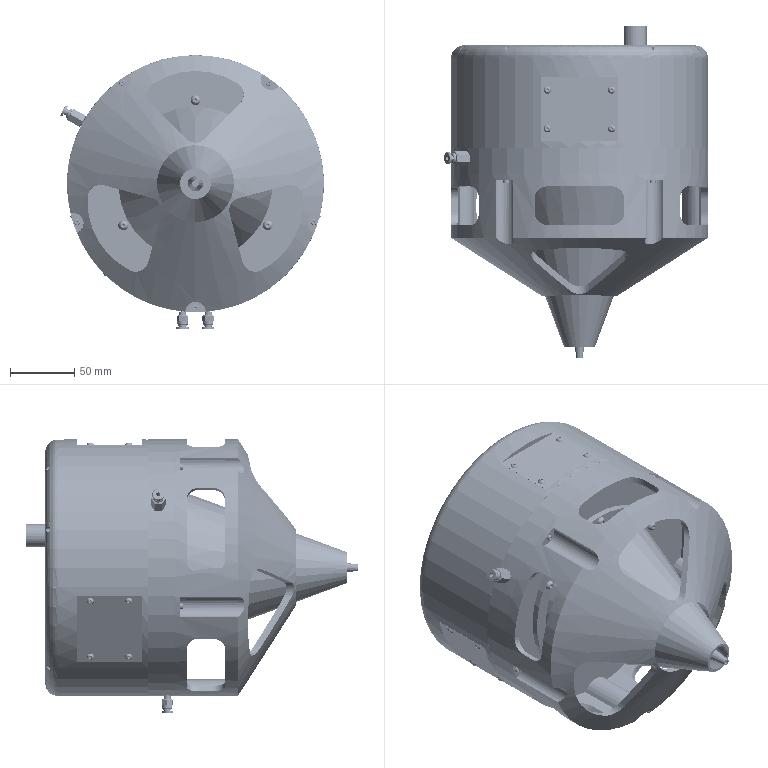Assembly | SolidWorks | mm | 111 component files | 112 solids | 5909 faces | box 205.4 x 258.5 x 213 mm | volume 1663403 mm3 | plane 2916 | cylinder 2290 | cone 400 | torus 202 | sphere 60 | spline 41 | commonest cylinder face diameters 5 x522 3 x431 7 x304 2 x192 4 x140 2.4 x66 20 x51 6 x38
Bill of materials:
AirSupplyPneumaticQuickConnectorM5 | 1 |  | Axisymmetric multi-diameter body around a hexagonal prism section. On one side of the hex is a short neck with ring/groove steps, then a thin round disk-like flange that has a central bore. On the other side is a smaller cylindrical spigot with a chamfered end and a small central hole.
CoolingPlateCover | 1 |  | Thin plain solid circular disc.
CornerCubePrism | 1 |  | Solid cylinder with one flat end and the other end cut by two inclined planes forming a ridged, roof-like end; one radial hole that appears threaded in the cylindrical wall.
CornerCubePrismCoolingPlate | 1 |  | Flanged hub: triangular plate with rounded corners and three corner through-holes, with a cylindrical boss on one side; the boss has small radial holes in its wall.
FocusingLens | 3 |  | Plain solid circular disc, thicker than a thin shim.
FocusingLensHolder | 3 |  | Square flat plate with slightly rounded corners, a large central through-hole and four smaller corner through-holes.
GB_SOCKET_TYPE7 M3X6-N | 24 |  | Headed pin: a domed (round-top) head on a plain cylindrical shank with a flat end.
GB_SOCKET_TYPE7 M4X10-N | 6 |  | Button/dome-head fastener shape with a hexagonal socket recess in the head and a plain cylindrical shank.
GB_FASTENER_SCREWS_HSHCS M2.5X6-N | 3 |  | Short cylindrical-head fastener shape: a tall round head with rounded top edge on a plain cylindrical shank with a chamfered end.
GB_FASTENER_SCREWS_HSHCS M2.5X10-N | 5 |  | Socket-head cap screw-like shape: a cylindrical head with a hexagonal socket and a cone-shaped bottom, on a long plain cylindrical shank.
GB_FASTENER_SCREWS_HSHCS M2X8-N | 2 |  | Cylindrical-head fastener shape: a round head with radiused top edge on a long plain cylindrical shank with a chamfered tip.
LaserWorkingHeadCoreComponent | 1 |  | Large circular plate with a stepped edge (reduced-diameter step on one face), three rectangular through-cutouts spaced around the center, and many small holes in the face plus at least one radial hole in the rim.
LaserWorkingHeadCover(Upper)2 | 3 |  | Flat rectangular plate with four through-holes near the corners.
LaserWorkingHeadHood(Lower) | 1 |  | Open, skeletal cup-shaped frame: cylindrical ring wall with several rounded slots, joined to a conical section that tapers to a central circular opening, with three spokes separating three large rounded windows.
Nozzle1 | 1 |  | Flanged tube: three-lobed flange with three through-holes at one end of a long cylindrical tube, with an angled wedge-like fin projecting from one side of the tube; the far end face shows a central bore surrounded by small holes.
Nozzle2 | 1 |  | Flanged tapered nozzle-like body: circular flange with three through-holes, then a cylindrical section and a conical taper ending in a small tip with a through bore; the flange side shows an internal conical cavity.
NozzleGasket1 | 1 |  | Thin three-lobed flat ring with a large central hole and a through-hole in each of the three lobes.
NozzleGasket2 | 1 |  | Flat circular ring (annular plate) with a large central hole and three equally spaced small through-holes.
Reflector | 3 |  | Solid short cylinder with one end cut off at an angle, so it ends in a wedge. A radial hole in the side wall appears threaded and has a counterbore or spot face around it.
Slider2 | 3 |  | Rectangular prismatic block with internal cylindrical passages. One passage has a stepped diameter and conical (drill-point-like) ends. The block also has a shallow groove across one face and small V-shaped notches with rounded bottoms on its edges.
Slider | 3 |  | Flat rectangular plate with rounded corners and two round through-holes. Shallow notches or grooves cross the long edges near each end. A V-shaped tab with a semicircular cutout sticks out from one long edge, and a small slot is cut into one side.
Slider3 | 3 |  | Rectangular block with a long groove on top that has angled sides, plus a narrow slit. A V-notch with a round bottom is cut into the end face. Underneath, a cylindrical or rounded boss is split by a central slot.
SliderNut1 | 3 |  | Knurled cylindrical head joined to a smaller smooth cylindrical shank. A central bore runs axially through both, and a small cross-hole passes through the shank wall.
SliderNut2 | 3 |  | Knurled cylindrical head with a smooth, smaller cylindrical shank. The visible flat end faces look solid, with no bore.
SliderScrew1 | 3 |  | Stepped cylindrical pin. A short reduced-diameter pilot is at one end, followed by a main body interrupted by a narrow circumferential groove. The other end is flat.
SliderScrew2 | 3 |  | Stepped cylindrical pin with a narrow necked groove between two equal-diameter sections. One end has a smaller-diameter cylindrical spigot.
T-Joint | 1 |  | Tubular multi-port body with three or more cylindrical ports and stepped collars at the port ends. Small ring-shaped bosses with through-holes sit beside the branch.
UpperHousing | 1 |  | Thin-walled cylindrical shell or drum with one closed end face. The end face has a large central hole, a bolt-hole pattern and small holes around a raised rim. Rectangular windows and recessed pads with small holes are cut into the side wall.
WaterPipe1 | 1 |  | Slender solid round rod bent into a curve of roughly a half-circle to three-quarters of a circle, with a short straight end section. The ends are rounded.
WaterPipe2 | 1 |  | Hollow round tube bent into a 3D path with straight runs joined by a sharp-ish bend and a roughly 90-degree radiused bend. Both ends are open and cut square.
WaterPipe3 | 1 |  | Thin-walled round tube bent into a multi-bend, roughly V/hook-shaped path, shown as two tube segments separated by a small gap along one straight run.
WaterPipe4 | 1 |  | Round tube or rod bent in three dimensions with several bends, including a sharp near-90-degree turn to one end leg.
WaterPipe5 | 1 |  | Short straight hollow cylinder (sleeve or tube section) with plain square-cut ends.
WaterPipe6 | 1 |  | Hollow round tube bent into an offset/Z-like shape: straight end leg, a long angled run, and a second bend into a short end leg.
WaterPipe7 | 1 |  | Relatively thick-walled hollow tube with several bends, including an S-curve and roughly right-angle turns.
WaterQuickConnector | 12 |  | Axially stepped turned-style body: thin circular flange disc with a large bore at one end, a grooved cylindrical collar, a hexagonal wrench-flat section, then stepped smaller cylindrical spigots ending in a small-bore tip.
WireConnectorBlock1 | 1 |  | Flat obround (stadium-shaped) plate with one large central through-hole and two smaller through-holes, one near each rounded end.
WireFeedingConnector | 1 |  | Stepped cylinder: a large-diameter main cylinder with a smaller, coaxial hollow boss sticking out from one end face, and a small central through-bore.
WireFeedingHose | 1 |  | Long, slender hollow tube that is mostly straight, with a gentle bend near one end.
WireFeedingNozzle | 1 |  | Hollow, round, spigot-like body: a long tapered section narrowing to a rounded tip, a short necked transition, a raised cylindrical collar, and a straight cylindrical end section.
WireFeedingTube | 1 |  | Hollow stepped cylindrical shaft or spacer: a long central section of larger diameter with shorter reduced-diameter sections at both ends, and a central through-bore.
WorkingHeadLowerCover | 1 |  | Thin-walled hollow cone (funnel- or hopper-like) with a flat annular flange at the large end and an open small end.
Y-Joint | 1 |  | Y-shaped tubular body. A single cylindrical branch at one end splits into two parallel cylindrical branches side by side at the other end. Every branch ends in a hollow round port with a flanged collar. A short cylindrical boss with a through-hole sits at the junction, with its hole running at right angles to the branch axes.
Mates:
1. concentric | LaserWorkingHeadCoreComponent-1 face at (-15.981, 4.506, 234.566) dir (0, 1, 0) r 2 | Slider-3 face at (-15.981, 15.849, 234.566) dir (0, 1, 0) r 1.65
2. concentric | LaserWorkingHeadCoreComponent-1 face at (4.019, 4.506, 234.566) dir (0, 1, 0) r 2 | Slider-3 face at (4.019, 15.849, 234.566) dir (0, 1, 0) r 1.65
3. coincident | LaserWorkingHeadCoreComponent-1 face at (-5.981, 10.506, 160) dir (0, 1, 0) | Slider-3 face at (-5.981, 10.506, 234.566) dir (0, -1, 0)
4. coincident | LaserWorkingHeadCoreComponent-1 face at (-5.981, 10.506, 160) dir (0, 1, 0) | Slider-4 face at (58.596, 10.506, 122.717) dir (0, -1, 0)
5. coincident | LaserWorkingHeadCoreComponent-1 face at (-5.981, 10.506, 160) dir (0, 1, 0) | Slider-5 face at (-70.557, 10.506, 122.717) dir (0, -1, 0)
6. concentric | Slider2-2 face at (68.988, 19.006, 116.717) dir (-0.866, 0, 0.5) r 1.5 | SliderScrew1-2 face at (46.471, 19.006, 129.717) dir (0.866, 0, -0.5) r 1.5
7. concentric | Slider2-3 face at (-5.981, 19.006, 246.566) dir (0, 0, -1) r 1.5 | SliderScrew1-3 face at (-5.981, 19.006, 220.566) dir (0, 0, 1) r 1.5
8. concentric | Slider2-3 face at (-20.981, 33.561, 233.566) dir (1, 0, 0) r 1.5 | Slider3-3 face at (9.019, 33.561, 233.566) dir (-1, 0, 0) r 1.5
9. coincident | Slider2-3 face at (-5.981, 19.006, 236.566) dir (0, 0, -1) | Slider3-3 face at (9.019, 40.533, 236.566) dir (0, 0, 1)
10. concentric | Slider3-6 face at (-77.191, 33.561, 136.207) dir (0.5, 0, -0.866) r 1.5 | Slider2-6 face at (-62.191, 33.561, 110.226) dir (-0.5, 0, 0.866) r 1.5
11. coincident | Slider3-6 face at (-79.789, 40.533, 134.707) dir (-0.866, 0, -0.5) | Slider2-6 face at (-72.289, 19.006, 121.717) dir (0.866, 0, 0.5)
12. concentric | Slider2-6 face at (-80.95, 19.006, 116.717) dir (0.866, 0, 0.5) r 1.5 | SliderScrew1-1 face at (-58.433, 19.006, 129.717) dir (-0.866, 0, -0.5) r 1.5
13. concentric | Slider2-2 face at (65.23, 33.561, 136.207) dir (-0.5, 0, -0.866) r 1.5 | Slider3-7 face at (50.23, 33.561, 110.226) dir (0.5, 0, 0.866) r 1.5
14. coincident | Slider2-2 face at (60.328, 19.006, 121.717) dir (-0.866, 0, 0.5) | Slider3-7 face at (52.828, 40.533, 108.726) dir (0.866, 0, -0.5)
15. concentric | SliderScrew1-1 face at (-83.115, 19.006, 115.467) dir (0.866, 0, 0.5) r 1 | SliderNut1-1 face at (-83.115, 19.006, 115.467) dir (0.866, 0, 0.5) r 1
16. coincident | SliderScrew1-1 face at (-80.95, 19.006, 116.717) dir (-0.866, 0, -0.5) | SliderNut1-1 face at (-80.435, 20.722, 115.826) dir (0.866, 0, 0.5)
17. concentric | SliderScrew1-2 face at (71.153, 19.006, 115.467) dir (-0.866, 0, 0.5) r 1 | SliderNut1-2 face at (71.153, 19.006, 115.467) dir (-0.866, 0, 0.5) r 1
18. coincident | SliderScrew1-2 face at (68.988, 19.006, 116.717) dir (0.866, 0, -0.5) | SliderNut1-2 face at (68.893, 20.997, 116.552) dir (-0.866, 0, 0.5)
19. concentric | Slider2-2 axis at (68.988, 19.006, 116.717) dir (-0.866, 0, 0.5) | SliderScrew1-2 face at (58.271, 19.006, 122.904) dir (-0.866, 0, 0.5) r 1
20. coincident | Slider-4 face at (61.488, 20.506, 103.726) dir (0.866, 0, -0.5) | SliderNut1-2 edge at (68.988, 19.006, 116.717) dir (-0.866, 0, 0.5) r 2
21. coincident | Slider-5 face at (-73.45, 20.506, 103.726) dir (-0.866, 0, -0.5) | SliderNut1-1 face at (-80.435, 20.722, 115.826) dir (0.866, 0, 0.5)
22. concentric | SliderScrew1-3 face at (-5.981, 19.006, 249.066) dir (0, 0, -1) r 1 | SliderNut1-3 face at (-5.981, 19.006, 249.066) dir (0, 0, -1) r 1
23. coincident | SliderScrew1-3 face at (-5.981, 19.006, 246.566) dir (0, 0, 1) | SliderNut1-3 face at (-4.046, 18.501, 246.566) dir (0, 0, -1)
24. concentric | SliderScrew1-3 face at (-5.981, 19.006, 234.191) dir (0, 0, -1) r 1 | Slider2-3 face at (-5.981, 19.006, 246.566) dir (0, 0, -1) r 1.5
25. coincident | Slider-3 face at (9.019, 20.506, 246.566) dir (0, 0, 1) | SliderNut1-3 face at (-4.046, 18.501, 246.566) dir (0, 0, -1)
26. concentric | SliderScrew2-1 face at (12.019, 33.561, 233.566) dir (-1, 0, 0) r 0.8 | SliderNut2-1 face at (12.519, 33.561, 233.566) dir (-1, 0, 0) r 1
27. coincident | SliderScrew2-1 face at (9.019, 33.561, 233.566) dir (1, 0, 0) | SliderNut2-1 face at (9.019, 33.561, 233.566) dir (-1, 0, 0)
28. concentric | Slider3-3 face at (9.019, 33.561, 233.566) dir (-1, 0, 0) r 1.5 | SliderScrew2-1 face at (-6.731, 33.561, 233.566) dir (1, 0, 0) r 0.8
29. coincident | Slider3-3 face at (9.019, 33.561, 233.566) dir (1, 0, 0) | SliderNut2-1 face at (9.019, 33.561, 233.566) dir (-1, 0, 0)
30. concentric | SliderScrew2-2 face at (-78.691, 33.561, 138.805) dir (0.5, 0, -0.866) r 0.8 | SliderNut2-2 face at (-78.941, 33.561, 139.238) dir (0.5, 0, -0.866) r 1
31. coincident | SliderScrew2-2 face at (-77.191, 33.561, 136.207) dir (-0.5, 0, 0.866) | SliderNut2-2 face at (-77.191, 33.561, 136.207) dir (0.5, 0, -0.866)
32. concentric | Slider3-6 face at (-77.191, 33.561, 136.207) dir (0.5, 0, -0.866) r 1.5 | SliderScrew2-2 face at (-69.316, 33.561, 122.567) dir (-0.5, 0, 0.866) r 0.8
33. coincident | Slider3-6 face at (-77.191, 33.561, 136.207) dir (-0.5, 0, 0.866) | SliderNut2-2 face at (-77.191, 33.561, 136.207) dir (0.5, 0, -0.866)
34. concentric | SliderScrew2-3 face at (48.73, 33.561, 107.628) dir (0.5, 0, 0.866) r 0.8 | SliderNut2-3 face at (48.48, 33.561, 107.195) dir (0.5, 0, 0.866) r 1
35. coincident | SliderScrew2-3 face at (50.23, 33.561, 110.226) dir (-0.5, 0, -0.866) | SliderNut2-3 face at (50.23, 33.561, 110.226) dir (0.5, 0, 0.866)
36. concentric | Slider3-7 face at (50.23, 33.561, 110.226) dir (0.5, 0, 0.866) r 1.5 | SliderScrew2-3 face at (58.105, 33.561, 123.866) dir (-0.5, 0, -0.866) r 0.8
37. coincident | Slider3-7 face at (50.23, 33.561, 110.226) dir (-0.5, 0, -0.866) | SliderNut2-3 face at (50.23, 33.561, 110.226) dir (0.5, 0, 0.866)
38. concentric | Nozzle1-1 face at (-19.837, -106.495, 152) dir (0, 1, 0) r 1.5 | NozzleGasket1-1 face at (-19.837, -9.493, 152) dir (0, -1, 0) r 1.5
39. coincident | Nozzle1-1 face at (-23.301, -11.494, 150) dir (0, 1, 0) | NozzleGasket1-1 face at (-5.981, -11.494, 160) dir (0, -1, 0)
40. concentric | Nozzle1-1 face at (-5.981, -106.495, 176) dir (0, 1, 0) r 1.5 | NozzleGasket1-1 face at (-5.981, -9.493, 176) dir (0, -1, 0) r 1.5
41. coincident | LaserWorkingHeadCoreComponent-1 face at (-5.981, -9.494, 160) dir (0, -1, 0) | NozzleGasket1-1 face at (-5.981, -9.494, 160) dir (0, 1, 0)
42. concentric | LaserWorkingHeadCoreComponent-1 face at (-5.981, -2.494, 176) dir (0, -1, 0) r 1.5 | Nozzle1-1 face at (-5.981, -106.495, 176) dir (0, 1, 0) r 1.5
43. concentric | LaserWorkingHeadCoreComponent-1 face at (7.876, -2.494, 152) dir (0, -1, 0) r 1.5 | Nozzle1-1 face at (7.876, -106.495, 152) dir (0, 1, 0) r 1.5
44. concentric | Nozzle1-1 face at (-5.981, -101.494, 168) dir (0, -1, 0) r 1 | NozzleGasket2-1 face at (-5.981, -106.494, 168) dir (0, -1, 0) r 1
45. concentric | Nozzle1-1 face at (0.9473, -101.494, 156) dir (0, -1, 0) r 1 | NozzleGasket2-1 face at (0.9473, -106.494, 156) dir (0, -1, 0) r 1
46. coincident | Nozzle1-1 face at (-5.981, -106.494, 160) dir (0, -1, 0) | NozzleGasket2-1 face at (-5.981, -106.494, 160) dir (0, 1, 0)
47. concentric | Nozzle1-1 face at (-5.981, -86.494, 160) dir (0, -1, 0) r 2.75 | WireFeedingNozzle-1 face at (-5.981, -144.495, 160) dir (0, 1, 0) r 1.5
48. coincident | NozzleGasket2-1 face at (-5.981, -107.994, 160) dir (0, -1, 0) | WireFeedingNozzle-1 face at (-2.126, -107.994, 158.211) dir (0, 1, 0)
49. concentric | NozzleGasket2-1 face at (-12.909, -106.494, 156) dir (0, -1, 0) r 1 | Nozzle2-1 face at (-12.909, -152.995, 156) dir (0, 1, 0) r 1
50. concentric | NozzleGasket2-1 face at (-5.981, -106.494, 168) dir (0, -1, 0) r 1 | Nozzle2-1 face at (-5.981, -152.995, 168) dir (0, 1, 0) r 1
51. coincident | NozzleGasket2-1 face at (-5.981, -107.994, 160) dir (0, -1, 0) | Nozzle2-1 face at (2.679, -107.994, 155) dir (0, 1, 0)
52. concentric | LaserWorkingHeadCoreComponent-1 face at (40.271, 10.506, 179.775) dir (0, 1, 0) r 1 | WireConnectorBlock1-1 face at (40.271, 20.506, 179.775) dir (0, -1, 0) r 1
53. concentric | LaserWorkingHeadCoreComponent-1 face at (34.271, 10.506, 190.168) dir (0, 1, 0) r 1 | WireConnectorBlock1-1 face at (34.271, 20.506, 190.168) dir (0, -1, 0) r 1
54. coincident | LaserWorkingHeadCoreComponent-1 face at (-5.981, 15.506, 160) dir (0, 1, 0) | WireConnectorBlock1-1 face at (37.271, 15.506, 184.972) dir (0, -1, 0)
55. concentric | LaserWorkingHeadCoreComponent-1 face at (-7.731, 2.506, 160.968) dir (-0.875, 0, 0.4841) r 2.5 | AirSupplyPneumaticQuickConnectorM5-2 axis at (-94.357, 2.506, 208.894) dir (0.875, 0, -0.4841)
56. tangent | LaserWorkingHeadCoreComponent-1 face at (-5.981, 15.506, 160) dir (0, -1, 0) r 100 | AirSupplyPneumaticQuickConnectorM5-2 face at (-91.24, 2.532, 212.463) dir (0.875, 0, -0.4841)
57. concentric | LaserWorkingHeadCoreComponent-1 face at (53.596, 4.506, 114.057) dir (0, 1, 0) r 2 | Slider-4 face at (53.596, 15.849, 114.057) dir (0, 1, 0) r 1.65
58. concentric | LaserWorkingHeadCoreComponent-1 face at (63.596, 4.506, 131.377) dir (0, 1, 0) r 2 | Slider-4 face at (63.596, 15.849, 131.377) dir (0, 1, 0) r 1.65
59. concentric | LaserWorkingHeadCoreComponent-1 face at (-75.557, 4.506, 131.377) dir (0, 1, 0) r 2 | Slider-5 face at (-75.557, 15.849, 131.377) dir (0, 1, 0) r 1.65
60. concentric | LaserWorkingHeadCoreComponent-1 face at (-65.557, 4.506, 114.057) dir (0, 1, 0) r 2 | Slider-5 face at (-65.557, 15.849, 114.057) dir (0, 1, 0) r 1.65
61. concentric | LaserWorkingHeadCoreComponent-1 face at (50.446, 2.506, 237.666) dir (0, 1, 0) r 2.5 | UpperHousing-1 face at (50.446, 90.507, 237.666) dir (0, -1, 0) r 2
62. concentric | LaserWorkingHeadCoreComponent-1 face at (85.321, 2.506, 189.666) dir (0, 1, 0) r 2.5 | UpperHousing-1 face at (85.321, 90.507, 189.666) dir (0, -1, 0) r 2
63. concentric | LaserWorkingHeadCoreComponent-1 face at (-62.408, 2.506, 237.666) dir (0, 1, 0) r 2.5 | UpperHousing-1 face at (-62.408, 90.507, 237.666) dir (0, -1, 0) r 2
64. coincident | LaserWorkingHeadCoreComponent-1 face at (-5.981, 10.506, 160) dir (0, 1, 0) | UpperHousing-1 face at (-5.981, 10.506, 160) dir (0, -1, 0)
65. concentric | UpperHousing-1 face at (37.32, 10.505, 185) dir (0, 1, 0) r 3.5 | WireFeedingConnector-1 face at (37.32, 109.006, 185) dir (0, 1, 0) r 1.5
66. coincident | UpperHousing-1 face at (-5.981, 90.506, 160) dir (0, 1, 0) | WireFeedingConnector-1 face at (36.423, 90.506, 188.383) dir (0, -1, 0)
67. concentric | WireFeedingConnector-1 face at (37.32, 109.006, 185) dir (0, 1, 0) r 1.5 | WireFeedingTube-1 face at (37.32, 12.531, 185) dir (0, -1, 0) r 1.5
68. coincident | WireFeedingConnector-1 face at (36.936, 85.506, 186.45) dir (0, -1, 0) | WireFeedingTube-1 face at (39.434, 85.506, 186.336) dir (0, 1, 0)
69. concentric | FocusingLensHolder-1 face at (-5.981, 12.506, 205.812) dir (0, 1, 0) r 10 | FocusingLens-1 face at (-5.981, 15.506, 205.812) dir (0, -1, 0) r 10
70. coincident | FocusingLensHolder-1 face at (-5.981, 12.506, 205.812) dir (0, 1, 0) | FocusingLens-1 face at (-5.981, 12.506, 205.812) dir (0, -1, 0)
71. concentric | FocusingLensHolder-2 face at (33.693, 12.506, 137.094) dir (0, 1, 0) r 10 | FocusingLens-2 face at (33.693, 15.506, 137.094) dir (0, -1, 0) r 10
72. coincident | FocusingLensHolder-2 face at (33.693, 12.506, 137.094) dir (0, 1, 0) | FocusingLens-2 face at (33.693, 12.506, 137.094) dir (0, -1, 0)
73. concentric | FocusingLensHolder-3 face at (-45.655, 12.506, 137.094) dir (0, 1, 0) r 10 | FocusingLens-3 face at (-45.655, 15.506, 137.094) dir (0, -1, 0) r 10
74. coincident | FocusingLensHolder-3 face at (-45.655, 12.506, 137.094) dir (0, 1, 0) | FocusingLens-3 face at (-45.655, 12.506, 137.094) dir (0, -1, 0)
75. concentric | LaserWorkingHeadCoreComponent-1 face at (-21.553, 6.506, 151.01) dir (0, 1, 0) r 1.5 | CornerCubePrismCoolingPlate-1 face at (-21.553, 15.506, 151.01) dir (0, -1, 0) r 1.5
76. concentric | LaserWorkingHeadCoreComponent-1 face at (-5.981, 6.506, 177.981) dir (0, 1, 0) r 1.5 | CornerCubePrismCoolingPlate-1 face at (-5.981, 15.506, 177.981) dir (0, -1, 0) r 1.5
77. coincident | LaserWorkingHeadCoreComponent-1 face at (-5.981, 11.506, 177.981) dir (0, 1, 0) | CornerCubePrismCoolingPlate-1 face at (-5.981, 11.506, 177.981) dir (0, -1, 0)
78. concentric | Slider3-7 face at (50.811, 23.56, 127.234) dir (0, 1, 0) r 1 | Reflector-5 face at (50.811, 39.061, 127.234) dir (0, 1, 0) r 1
79. coincident | Slider3-7 face at (45.899, 23.561, 112.726) dir (-0.866, 0, 0.5) | Reflector-5 face at (53.409, 33.561, 125.734) dir (0.866, 0, -0.5)
80. concentric | Slider3-7 face at (48.213, 33.561, 128.734) dir (0.866, 0, -0.5) r 7.5 | Reflector-5 face at (31.759, 33.561, 138.234) dir (0.866, 0, -0.5) r 7.5
81. concentric | Slider3-6 face at (-60.155, 33.561, 128.699) dir (-0.866, 0, -0.5) r 7.5 | Reflector-6 face at (-43.7, 33.561, 138.199) dir (-0.866, 0, -0.5) r 7.5
82. concentric | Slider3-6 face at (-62.753, 23.56, 127.199) dir (0, 1, 0) r 1 | Reflector-6 face at (-62.753, 39.061, 127.199) dir (0, 1, 0) r 1
83. concentric | Slider3-3 face at (-6.001, 33.561, 222.566) dir (0, 0, 1) r 7.5 | Reflector-4 face at (-6.001, 33.561, 203.566) dir (0, 0, 1) r 7.5
84. concentric | Slider3-3 face at (-6.001, 23.56, 225.566) dir (0, 1, 0) r 1 | Reflector-4 face at (-6.001, 39.061, 225.566) dir (0, 1, 0) r 1
85. concentric | Slider2-2 face at (68.988, 19.006, 116.717) dir (-0.866, 0, 0.5) r 1.5 | SliderScrew1-2 face at (46.471, 19.006, 129.717) dir (0.866, 0, -0.5) r 1.5
86. coincident | Slider-4 face at (61.488, 20.506, 103.726) dir (0.866, 0, -0.5) | Slider2-2 face at (68.988, 19.006, 116.717) dir (0.866, 0, -0.5)
87. coincident | Slider-5 face at (-73.45, 20.506, 103.726) dir (-0.866, 0, -0.5) | Slider2-6 face at (-80.95, 19.006, 116.717) dir (-0.866, 0, -0.5)
88. coincident | Slider-3 face at (9.019, 20.506, 246.566) dir (0, 0, 1) | Slider2-3 face at (-5.981, 19.006, 246.566) dir (0, 0, 1)
89. parallel | Slider-3 face at (-20.981, 15.849, 222.566) dir (0, 1, 0) | Slider2-3 face at (-20.981, 16.006, 246.566) dir (0, -1, 0)
90. coincident | Slider2-3 face at (-20.981, 46.006, 246.566) dir (-1, 0, 0) | Slider3-3 face at (-20.981, 33.561, 233.566) dir (-1, 0, 0)
91. parallel | Slider-4 face at (55.703, 15.849, 141.707) dir (0, 1, 0) | Slider2-2 face at (76.488, 16.006, 129.707) dir (0, -1, 0)
92. coincident | Slider2-2 face at (76.488, 46.006, 129.707) dir (0.5, 0, 0.866) | Slider3-7 face at (65.23, 33.561, 136.207) dir (0.5, 0, 0.866)
93. parallel | Slider-5 face at (-88.45, 15.849, 129.707) dir (0, 1, 0) | Slider2-6 face at (-83.7, 16.006, 121.48) dir (0, -1, 0)
94. coincident | Slider3-6 face at (-77.191, 33.561, 136.207) dir (-0.5, 0, 0.866) | Slider2-6 face at (-88.45, 46.006, 129.707) dir (-0.5, 0, 0.866)
95. coincident | Reflector-6 face at (-64.954, 33.561, 134.012) dir (-0.5, 0, 0.866) | WaterQuickConnector-1 face at (-64.954, 36.211, 134.012) dir (0.5, 0, -0.866)
96. parallel | Slider3-6 face at (-72.861, 23.561, 138.707) dir (0.866, 0, 0.5) | WaterQuickConnector-1 face at (-66.826, 32.561, 145.055) dir (0.866, 0, 0.5)
97. coincident | Reflector-6 face at (-57.954, 33.561, 121.887) dir (0.5, 0, -0.866) | WaterQuickConnector-2 face at (-57.954, 30.911, 121.887) dir (-0.5, 0, 0.866)
98. parallel | Slider3-6 face at (-72.861, 23.561, 138.707) dir (0.866, 0, 0.5) | WaterQuickConnector-2 face at (-49.326, 34.561, 114.744) dir (0.866, 0, 0.5)
99. coincident | Reflector-5 face at (46.012, 33.561, 121.922) dir (-0.5, 0, -0.866) | WaterQuickConnector-4 face at (46.012, 36.211, 121.922) dir (0.5, 0, 0.866)
100. parallel | Slider3-7 face at (45.899, 23.561, 112.726) dir (-0.866, 0, 0.5) | WaterQuickConnector-4 face at (37.385, 32.561, 114.779) dir (-0.866, 0, 0.5)
101. coincident | Reflector-5 face at (53.012, 33.561, 134.046) dir (0.5, 0, 0.866) | WaterQuickConnector-6 face at (53.012, 30.911, 134.046) dir (-0.5, 0, -0.866)
102. parallel | Slider3-7 face at (45.899, 23.561, 112.726) dir (-0.866, 0, 0.5) | WaterQuickConnector-6 face at (54.885, 34.561, 145.09) dir (-0.866, 0, 0.5)
103. concentric | Reflector-4 face at (1.5, 33.561, 224.066) dir (-1, 0, 0) r 1.5 | WaterQuickConnector-8 face at (47.999, 33.561, 224.066) dir (1, 0, 0) r 1.5
104. coincident | Reflector-4 face at (0.9989, 33.561, 224.066) dir (1, 0, 0) | WaterQuickConnector-8 face at (0.9989, 36.211, 224.066) dir (-1, 0, 0)
105. parallel | Slider3-3 face at (9.019, 23.561, 228.566) dir (0, 0, -1) | WaterQuickConnector-8 face at (11.499, 32.561, 220.166) dir (0, 0, -1)
106. coincident | Reflector-4 face at (-13.001, 33.561, 224.066) dir (-1, 0, 0) | WaterQuickConnector-10 face at (-13.001, 30.911, 224.066) dir (1, 0, 0)
107. parallel | Slider3-3 face at (9.019, 23.561, 228.566) dir (0, 0, -1) | WaterQuickConnector-10 face at (-23.501, 34.561, 220.166) dir (0, 0, -1)
108. concentric | WaterQuickConnector-6 face at (76.512, 33.561, 174.75) dir (0.5, 0, 0.866) r 2 | WaterPipe1-2 face at (54.985, 33.561, 137.464) dir (0.5, 0, 0.866) r 2
109. concentric | WaterQuickConnector-8 face at (47.999, 33.561, 224.066) dir (1, 0, 0) r 2 | WaterPipe1-2 face at (18.383, 33.561, 224.066) dir (-1, 0, 0) r 2
110. concentric | WaterQuickConnector-14 face at (-5.981, 20.506, 102) dir (0, 0, -1) r 1.5 | CornerCubePrismCoolingPlate-1 face at (-5.981, 20.506, 152.2) dir (0, 0, -1) r 1.5
111. concentric | LaserWorkingHeadCoreComponent-1 face at (4.019, -4.494, 85) dir (0, 0, -1) r 1.5 | WaterQuickConnector-18 face at (4.019, -4.494, 13) dir (0, 0, -1) r 1.5
112. tangent | LaserWorkingHeadCoreComponent-1 face at (-5.981, 15.506, 160) dir (0, -1, 0) r 100 | WaterQuickConnector-18 face at (6.467, -3.479, 60) dir (0, 0, 1)
113. concentric | LaserWorkingHeadCoreComponent-1 face at (-15.981, -4.494, 85) dir (0, 0, -1) r 1.5 | WaterQuickConnector-19 face at (-15.981, -4.494, 13) dir (0, 0, -1) r 1.5
114. tangent | LaserWorkingHeadCoreComponent-1 face at (-5.981, 15.506, 160) dir (0, -1, 0) r 100 | WaterQuickConnector-19 face at (-13.533, -3.479, 60) dir (0, 0, 1)
115. coincident | LaserWorkingHeadCoreComponent-1 face at (-5.981, 10.506, 160) dir (0, 1, 0) | FocusingLensHolder-2 face at (33.693, 10.506, 137.094) dir (0, -1, 0)
116. coincident | LaserWorkingHeadCoreComponent-1 face at (-5.981, 10.506, 160) dir (0, 1, 0) | FocusingLensHolder-3 face at (-45.655, 10.506, 137.094) dir (0, -1, 0)
117. coincident | LaserWorkingHeadCoreComponent-1 face at (-5.981, 10.506, 160) dir (0, 1, 0) | FocusingLensHolder-1 face at (-5.981, 10.506, 205.812) dir (0, -1, 0)
118. concentric | CornerCubePrismCoolingPlate-1 face at (-21.553, 15.506, 151.01) dir (0, -1, 0) r 1.5 | hexagon socket head cap screws gb-1 face at (-21.553, 7.106, 151.01) dir (0, 1, 0) r 1.25
119. coincident | CornerCubePrismCoolingPlate-1 face at (-21.553, 13.106, 151.01) dir (0, 1, 0) | hexagon socket head cap screws gb-1 face at (-21.553, 13.106, 151.01) dir (0, -1, 0)
120. concentric | CornerCubePrismCoolingPlate-1 face at (-5.981, 15.506, 177.981) dir (0, -1, 0) r 1.5 | hexagon socket head cap screws gb-2 face at (-5.981, 7.106, 177.981) dir (0, 1, 0) r 1.25
121. coincident | CornerCubePrismCoolingPlate-1 face at (-5.981, 13.106, 177.981) dir (0, 1, 0) | hexagon socket head cap screws gb-2 face at (-5.981, 13.106, 177.981) dir (0, -1, 0)
122. concentric | CornerCubePrismCoolingPlate-1 face at (9.591, 13.106, 151.01) dir (0, 1, 0) r 2.5 | hexagon socket head cap screws gb-3 face at (9.591, 7.106, 151.01) dir (0, 1, 0) r 1.25
123. coincident | CornerCubePrismCoolingPlate-1 face at (9.591, 13.106, 151.01) dir (0, 1, 0) | hexagon socket head cap screws gb-3 face at (9.591, 13.106, 151.01) dir (0, -1, 0)
124. concentric | FocusingLensHolder-2 face at (15.203, 15.506, 135.068) dir (0, -1, 0) r 1.7 | hexagon socket button head screws gb-1 face at (15.203, 9.506, 135.068) dir (0, 1, 0) r 1.5
125. coincident | FocusingLensHolder-2 face at (33.693, 15.506, 137.094) dir (0, 1, 0) | hexagon socket button head screws gb-1 face at (15.203, 15.506, 135.068) dir (0, -1, 0)
126. concentric | FocusingLensHolder-2 face at (26.203, 15.506, 154.121) dir (0, -1, 0) r 1.7 | hexagon socket button head screws gb-2 face at (26.203, 9.506, 154.121) dir (0, 1, 0) r 1.5
127. coincident | FocusingLensHolder-2 face at (33.693, 15.506, 137.094) dir (0, 1, 0) | hexagon socket button head screws gb-2 face at (26.203, 15.506, 154.121) dir (0, -1, 0)
128. concentric | FocusingLensHolder-2 face at (51.317, 15.506, 139.621) dir (0, -1, 0) r 1.7 | hexagon socket button head screws gb-3 face at (51.317, 9.506, 139.621) dir (0, 1, 0) r 1.5
129. coincident | FocusingLensHolder-2 face at (33.693, 15.506, 137.094) dir (0, 1, 0) | hexagon socket button head screws gb-3 face at (51.317, 15.506, 139.621) dir (0, -1, 0)
130. concentric | FocusingLensHolder-2 face at (40.317, 15.506, 120.568) dir (0, -1, 0) r 1.7 | hexagon socket button head screws gb-4 face at (40.317, 9.506, 120.568) dir (0, 1, 0) r 1.5
131. coincident | FocusingLensHolder-2 face at (33.693, 15.506, 137.094) dir (0, 1, 0) | hexagon socket button head screws gb-4 face at (40.317, 15.506, 120.568) dir (0, -1, 0)
132. concentric | FocusingLensHolder-3 face at (-27.164, 15.506, 135.068) dir (0, -1, 0) r 1.7 | hexagon socket button head screws gb-5 face at (-27.164, 9.506, 135.068) dir (0, 1, 0) r 1.5
133. coincident | FocusingLensHolder-3 face at (-45.655, 15.506, 137.094) dir (0, 1, 0) | hexagon socket button head screws gb-5 face at (-27.164, 15.506, 135.068) dir (0, -1, 0)
134. concentric | FocusingLensHolder-3 face at (-38.164, 15.506, 154.121) dir (0, -1, 0) r 1.7 | hexagon socket button head screws gb-6 face at (-38.164, 9.506, 154.121) dir (0, 1, 0) r 1.5
135. coincident | FocusingLensHolder-3 face at (-45.655, 15.506, 137.094) dir (0, 1, 0) | hexagon socket button head screws gb-6 face at (-38.164, 15.506, 154.121) dir (0, -1, 0)
136. concentric | FocusingLensHolder-3 face at (-63.279, 15.506, 139.621) dir (0, -1, 0) r 1.7 | hexagon socket button head screws gb-7 face at (-63.279, 9.506, 139.621) dir (0, 1, 0) r 1.5
137. coincident | FocusingLensHolder-3 face at (-45.655, 15.506, 137.094) dir (0, 1, 0) | hexagon socket button head screws gb-7 face at (-63.279, 15.506, 139.621) dir (0, -1, 0)
138. concentric | FocusingLensHolder-3 face at (-52.279, 15.506, 120.568) dir (0, -1, 0) r 1.7 | hexagon socket button head screws gb-8 face at (-52.279, 9.506, 120.568) dir (0, 1, 0) r 1.5
139. coincident | FocusingLensHolder-3 face at (-45.655, 15.506, 137.094) dir (0, 1, 0) | hexagon socket button head screws gb-8 face at (-52.279, 15.506, 120.568) dir (0, -1, 0)
140. concentric | FocusingLensHolder-1 face at (-16.981, 15.506, 190.812) dir (0, -1, 0) r 1.7 | hexagon socket button head screws gb-9 face at (-16.981, 9.506, 190.812) dir (0, 1, 0) r 1.5
141. coincident | FocusingLensHolder-1 face at (-5.981, 15.506, 205.812) dir (0, 1, 0) | hexagon socket button head screws gb-9 face at (-16.981, 15.506, 190.812) dir (0, -1, 0)
142. concentric | FocusingLensHolder-1 face at (5.019, 15.506, 190.812) dir (0, -1, 0) r 1.7 | hexagon socket button head screws gb-10 face at (5.019, 9.506, 190.812) dir (0, 1, 0) r 1.5
143. coincident | FocusingLensHolder-1 face at (-5.981, 15.506, 205.812) dir (0, 1, 0) | hexagon socket button head screws gb-10 face at (5.019, 15.506, 190.812) dir (0, -1, 0)
144. concentric | FocusingLensHolder-1 face at (-16.981, 15.506, 219.812) dir (0, -1, 0) r 1.7 | hexagon socket button head screws gb-11 face at (-16.981, 9.506, 219.812) dir (0, 1, 0) r 1.5
145. coincident | FocusingLensHolder-1 face at (-5.981, 15.506, 205.812) dir (0, 1, 0) | hexagon socket button head screws gb-11 face at (-16.981, 15.506, 219.812) dir (0, -1, 0)
146. concentric | FocusingLensHolder-1 face at (5.019, 15.506, 219.812) dir (0, -1, 0) r 1.7 | hexagon socket button head screws gb-12 face at (5.019, 9.506, 219.812) dir (0, 1, 0) r 1.5
147. coincident | FocusingLensHolder-1 face at (-5.981, 15.506, 205.812) dir (0, 1, 0) | hexagon socket button head screws gb-12 face at (5.019, 15.506, 219.812) dir (0, -1, 0)
148. concentric | WireConnectorBlock1-1 face at (34.271, 20.406, 190.168) dir (0, -1, 0) r 785.398 | hexagon socket head cap screws gb-4 face at (34.271, 12.506, 190.168) dir (0, 1, 0) r 1
149. coincident | WireConnectorBlock1-1 face at (37.271, 20.506, 184.972) dir (0, 1, 0) | hexagon socket head cap screws gb-4 face at (34.271, 20.506, 190.168) dir (0, -1, 0)
150. concentric | WireConnectorBlock1-1 face at (40.271, 20.406, 179.775) dir (0, -1, 0) r 785.398 | hexagon socket head cap screws gb-5 face at (40.271, 12.506, 179.775) dir (0, 1, 0) r 1
151. coincident | WireConnectorBlock1-1 face at (37.271, 20.506, 184.972) dir (0, 1, 0) | hexagon socket head cap screws gb-5 face at (40.271, 20.506, 179.775) dir (0, -1, 0)
152. coincident | UpperHousing-1 face at (-5.981, 10.506, 252) dir (0, 0, 1) | LaserWorkingHeadCover(Upper)2-4 face at (-5.981, 40.506, 252) dir (0, 0, -1)
153. concentric | UpperHousing-1 face at (19.019, 55.506, 59.999) dir (0, 0, 1) r 1.5 | LaserWorkingHeadCover(Upper)2-4 face at (19.019, 55.506, 255.5) dir (0, 0, -1) r 1.5
154. concentric | UpperHousing-1 face at (-30.981, 25.506, 59.999) dir (0, 0, 1) r 1.5 | LaserWorkingHeadCover(Upper)2-4 face at (-30.981, 25.506, 255.5) dir (0, 0, -1) r 1.5
155. coincident | UpperHousing-1 face at (73.693, 10.506, 114) dir (0.866, 0, -0.5) | LaserWorkingHeadCover(Upper)2-5 face at (73.693, 40.506, 114) dir (-0.866, 0, 0.5)
156. concentric | UpperHousing-1 face at (-136.783, 55.506, 206.651) dir (0.866, 0, -0.5) r 1.5 | LaserWorkingHeadCover(Upper)2-5 face at (64.225, 55.506, 90.599) dir (-0.866, 0, 0.5) r 1.5
157. concentric | UpperHousing-1 edge at (86.193, 25.506, 135.651) dir (0.866, 0, -0.5) r 1.5 | LaserWorkingHeadCover(Upper)2-5 face at (89.225, 25.506, 133.901) dir (-0.866, 0, 0.5) r 1.5
158. coincident | UpperHousing-1 face at (-85.655, 10.506, 114) dir (-0.866, 0, -0.5) | LaserWorkingHeadCover(Upper)2-7 face at (-85.655, 40.506, 114) dir (0.866, 0, 0.5)
159. concentric | UpperHousing-1 face at (99.822, 55.506, 249.953) dir (-0.866, 0, -0.5) r 1.5 | LaserWorkingHeadCover(Upper)2-7 face at (-101.186, 55.506, 133.901) dir (0.866, 0, 0.5) r 1.5
160. concentric | UpperHousing-1 face at (124.822, 25.506, 206.651) dir (-0.866, 0, -0.5) r 1.5 | LaserWorkingHeadCover(Upper)2-7 face at (-76.186, 25.506, 90.599) dir (0.866, 0, 0.5) r 1.5
161. concentric | LaserWorkingHeadCoreComponent-1 face at (-5.981, 15.506, 160) dir (0, -1, 0) r 100 | LaserWorkingHeadHood(Lower)-1 face at (-5.981, -109.494, 160) dir (0, 1, 0) r 100
162. coincident | LaserWorkingHeadCoreComponent-1 face at (-5.981, -9.494, 160) dir (0, -1, 0) | LaserWorkingHeadHood(Lower)-1 face at (-5.981, -9.494, 160) dir (0, 1, 0)
163. concentric | LaserWorkingHeadHood(Lower)-1 face at (-98.233, -9.494, 130.025) dir (0, -1, 0) r 1.5 | hexagon socket head cap screws gb-6 face at (-98.233, -4.494, 130.025) dir (0, -1, 0) r 1.25
164. coincident | LaserWorkingHeadHood(Lower)-1 face at (-101.087, -14.494, 129.098) dir (0, -1, 0) | hexagon socket head cap screws gb-6 face at (-98.233, -14.494, 130.025) dir (0, 1, 0)
165. concentric | LaserWorkingHeadHood(Lower)-1 face at (-62.996, -9.494, 238.475) dir (0, -1, 0) r 1.5 | hexagon socket head cap screws gb-7 face at (-62.996, -4.494, 238.475) dir (0, -1, 0) r 1.25
166. coincident | LaserWorkingHeadHood(Lower)-1 face at (-64.759, -14.494, 240.902) dir (0, -1, 0) | hexagon socket head cap screws gb-7 face at (-62.996, -14.494, 238.475) dir (0, 1, 0)
167. concentric | LaserWorkingHeadHood(Lower)-1 face at (-5.981, -9.494, 63) dir (0, -1, 0) r 1.5 | hexagon socket head cap screws gb-8 face at (-5.981, -4.494, 63) dir (0, -1, 0) r 1.25
168. coincident | LaserWorkingHeadHood(Lower)-1 face at (-5.981, -14.494, 60) dir (0, -1, 0) | hexagon socket head cap screws gb-8 face at (-5.981, -14.494, 63) dir (0, 1, 0)
169. concentric | LaserWorkingHeadHood(Lower)-1 face at (86.272, -9.494, 130.025) dir (0, -1, 0) r 1.5 | hexagon socket head cap screws gb-9 face at (86.272, -4.494, 130.025) dir (0, -1, 0) r 1.25
170. coincident | LaserWorkingHeadHood(Lower)-1 face at (89.125, -14.494, 129.098) dir (0, -1, 0) | hexagon socket head cap screws gb-9 face at (86.272, -14.494, 130.025) dir (0, 1, 0)
171. concentric | LaserWorkingHeadHood(Lower)-1 face at (51.034, -9.494, 238.475) dir (0, -1, 0) r 1.5 | hexagon socket head cap screws gb-10 face at (51.034, -4.494, 238.475) dir (0, -1, 0) r 1.25
172. coincident | LaserWorkingHeadHood(Lower)-1 face at (52.798, -14.494, 240.902) dir (0, -1, 0) | hexagon socket head cap screws gb-10 face at (51.034, -14.494, 238.475) dir (0, 1, 0)
173. concentric | LaserWorkingHeadCoreComponent-1 face at (-5.981, 15.506, 160) dir (0, -1, 0) r 100 | WorkingHeadLowerCover-1 face at (-5.981, -9.494, 160) dir (0, 1, 0) r 70
174. coincident | LaserWorkingHeadCoreComponent-1 face at (-5.981, -9.494, 160) dir (0, -1, 0) | WorkingHeadLowerCover-1 face at (54.641, -9.494, 125) dir (0, 1, 0)
175. concentric | LaserWorkingHeadCover(Upper)2-5 face at (89.225, 55.506, 133.901) dir (-0.866, 0, 0.5) r 1.5 | hexagon socket button head screws gb-13 face at (84.028, 55.506, 136.901) dir (0.866, 0, -0.5) r 1.5
176. coincident | LaserWorkingHeadCover(Upper)2-5 face at (76.725, 40.506, 112.25) dir (0.866, 0, -0.5) | hexagon socket button head screws gb-13 face at (89.225, 55.506, 133.901) dir (-0.866, 0, 0.5)
177. concentric | LaserWorkingHeadCover(Upper)2-5 face at (64.225, 55.506, 90.599) dir (-0.866, 0, 0.5) r 1.5 | hexagon socket button head screws gb-14 face at (59.028, 55.506, 93.599) dir (0.866, 0, -0.5) r 1.5
178. coincident | LaserWorkingHeadCover(Upper)2-5 face at (76.725, 40.506, 112.25) dir (0.866, 0, -0.5) | hexagon socket button head screws gb-14 face at (64.225, 55.506, 90.599) dir (-0.866, 0, 0.5)
179. concentric | LaserWorkingHeadCover(Upper)2-5 face at (64.225, 25.506, 90.599) dir (-0.866, 0, 0.5) r 1.5 | hexagon socket button head screws gb-15 face at (59.028, 25.506, 93.599) dir (0.866, 0, -0.5) r 1.5
180. coincident | LaserWorkingHeadCover(Upper)2-5 face at (76.725, 40.506, 112.25) dir (0.866, 0, -0.5) | hexagon socket button head screws gb-15 face at (64.225, 25.506, 90.599) dir (-0.866, 0, 0.5)
181. concentric | LaserWorkingHeadCover(Upper)2-5 face at (89.225, 25.506, 133.901) dir (-0.866, 0, 0.5) r 1.5 | hexagon socket button head screws gb-16 face at (84.028, 25.506, 136.901) dir (0.866, 0, -0.5) r 1.5
182. coincident | LaserWorkingHeadCover(Upper)2-5 face at (76.725, 40.506, 112.25) dir (0.866, 0, -0.5) | hexagon socket button head screws gb-16 face at (89.225, 25.506, 133.901) dir (-0.866, 0, 0.5)
183. concentric | LaserWorkingHeadCover(Upper)2-7 face at (-76.186, 55.506, 90.599) dir (0.866, 0, 0.5) r 1.5 | hexagon socket button head screws gb-17 face at (-70.99, 55.506, 93.599) dir (-0.866, 0, -0.5) r 1.5
184. coincident | LaserWorkingHeadCover(Upper)2-7 face at (-88.686, 40.506, 112.25) dir (-0.866, 0, -0.5) | hexagon socket button head screws gb-17 face at (-76.186, 55.506, 90.599) dir (0.866, 0, 0.5)
185. concentric | LaserWorkingHeadCover(Upper)2-7 face at (-101.186, 55.506, 133.901) dir (0.866, 0, 0.5) r 1.5 | hexagon socket button head screws gb-18 face at (-95.99, 55.506, 136.901) dir (-0.866, 0, -0.5) r 1.5
186. coincident | LaserWorkingHeadCover(Upper)2-7 face at (-88.686, 40.506, 112.25) dir (-0.866, 0, -0.5) | hexagon socket button head screws gb-18 face at (-101.186, 55.506, 133.901) dir (0.866, 0, 0.5)
187. concentric | LaserWorkingHeadCover(Upper)2-7 face at (-101.186, 25.506, 133.901) dir (0.866, 0, 0.5) r 1.5 | hexagon socket button head screws gb-19 face at (-95.99, 25.506, 136.901) dir (-0.866, 0, -0.5) r 1.5
188. coincident | LaserWorkingHeadCover(Upper)2-7 face at (-88.686, 40.506, 112.25) dir (-0.866, 0, -0.5) | hexagon socket button head screws gb-19 face at (-101.186, 25.506, 133.901) dir (0.866, 0, 0.5)
189. concentric | LaserWorkingHeadCover(Upper)2-7 face at (-76.186, 25.506, 90.599) dir (0.866, 0, 0.5) r 1.5 | hexagon socket button head screws gb-20 face at (-70.99, 25.506, 93.599) dir (-0.866, 0, -0.5) r 1.5
190. coincident | LaserWorkingHeadCover(Upper)2-7 face at (-88.686, 40.506, 112.25) dir (-0.866, 0, -0.5) | hexagon socket button head screws gb-20 face at (-76.186, 25.506, 90.599) dir (0.866, 0, 0.5)
191. concentric | LaserWorkingHeadCover(Upper)2-4 face at (19.019, 55.506, 255.5) dir (0, 0, -1) r 1.5 | hexagon socket button head screws gb-21 face at (19.019, 55.506, 249.5) dir (0, 0, 1) r 1.5
192. coincident | LaserWorkingHeadCover(Upper)2-4 face at (-5.981, 40.506, 255.5) dir (0, 0, 1) | hexagon socket button head screws gb-21 face at (19.019, 55.506, 255.5) dir (0, 0, -1)
193. concentric | LaserWorkingHeadCover(Upper)2-4 face at (19.019, 25.506, 255.5) dir (0, 0, -1) r 1.5 | hexagon socket button head screws gb-22 face at (19.019, 25.506, 249.5) dir (0, 0, 1) r 1.5
194. coincident | LaserWorkingHeadCover(Upper)2-4 face at (-5.981, 40.506, 255.5) dir (0, 0, 1) | hexagon socket button head screws gb-22 face at (19.019, 25.506, 255.5) dir (0, 0, -1)
195. concentric | LaserWorkingHeadCover(Upper)2-4 face at (-30.981, 55.506, 255.5) dir (0, 0, -1) r 1.5 | hexagon socket button head screws gb-23 face at (-30.981, 55.506, 249.5) dir (0, 0, 1) r 1.5
196. coincident | LaserWorkingHeadCover(Upper)2-4 face at (-5.981, 40.506, 255.5) dir (0, 0, 1) | hexagon socket button head screws gb-23 face at (-30.981, 55.506, 255.5) dir (0, 0, -1)
197. concentric | LaserWorkingHeadCover(Upper)2-4 face at (-30.981, 25.506, 255.5) dir (0, 0, -1) r 1.5 | hexagon socket button head screws gb-24 face at (-30.981, 25.506, 249.5) dir (0, 0, 1) r 1.5
198. coincident | LaserWorkingHeadCover(Upper)2-4 face at (-5.981, 40.506, 255.5) dir (0, 0, 1) | hexagon socket button head screws gb-24 face at (-30.981, 25.506, 255.5) dir (0, 0, -1)
199. concentric | LaserWorkingHeadCoreComponent-1 face at (50.311, -9.494, 192.5) dir (0, -1, 0) r 2 | WorkingHeadLowerCover-1 face at (50.311, -144.495, 192.5) dir (0, 1, 0) r 2.5
200. concentric | WorkingHeadLowerCover-1 face at (50.311, -144.495, 192.5) dir (0, 1, 0) r 2.5 | hexagon socket button head screws gb-25 face at (50.311, -4.494, 192.5) dir (0, -1, 0) r 2
201. coincident | WorkingHeadLowerCover-1 face at (45.981, -14.494, 130) dir (0, -1, 0) | hexagon socket button head screws gb-25 face at (50.311, -14.494, 192.5) dir (0, 1, 0)
202. concentric | WorkingHeadLowerCover-1 face at (50.311, -144.495, 127.5) dir (0, 1, 0) r 2.5 | hexagon socket button head screws gb-26 face at (50.311, -4.494, 127.5) dir (0, -1, 0) r 2
203. coincident | WorkingHeadLowerCover-1 face at (45.981, -14.494, 130) dir (0, -1, 0) | hexagon socket button head screws gb-26 face at (50.311, -14.494, 127.5) dir (0, 1, 0)
204. concentric | WorkingHeadLowerCover-1 face at (-5.981, -144.495, 95) dir (0, 1, 0) r 2.5 | hexagon socket button head screws gb-27 face at (-5.981, -4.494, 95) dir (0, -1, 0) r 2
205. coincident | WorkingHeadLowerCover-1 face at (45.981, -14.494, 130) dir (0, -1, 0) | hexagon socket button head screws gb-27 face at (-5.981, -14.494, 95) dir (0, 1, 0)
206. concentric | WorkingHeadLowerCover-1 face at (-62.273, -144.495, 127.5) dir (0, 1, 0) r 2.5 | hexagon socket button head screws gb-28 face at (-62.273, -4.494, 127.5) dir (0, -1, 0) r 2
207. coincident | WorkingHeadLowerCover-1 face at (45.981, -14.494, 130) dir (0, -1, 0) | hexagon socket button head screws gb-28 face at (-62.273, -14.494, 127.5) dir (0, 1, 0)
208. concentric | WorkingHeadLowerCover-1 face at (-62.273, -144.495, 192.5) dir (0, 1, 0) r 2.5 | hexagon socket button head screws gb-29 face at (-62.273, -4.494, 192.5) dir (0, -1, 0) r 2
209. coincident | WorkingHeadLowerCover-1 face at (45.981, -14.494, 130) dir (0, -1, 0) | hexagon socket button head screws gb-29 face at (-62.273, -14.494, 192.5) dir (0, 1, 0)
210. concentric | WorkingHeadLowerCover-1 face at (-5.981, -144.495, 225) dir (0, 1, 0) r 2.5 | hexagon socket button head screws gb-30 face at (-5.981, -4.494, 225) dir (0, -1, 0) r 2
211. coincident | WorkingHeadLowerCover-1 face at (45.981, -14.494, 130) dir (0, -1, 0) | hexagon socket button head screws gb-30 face at (-5.981, -14.494, 225) dir (0, 1, 0)
212. concentric | LaserWorkingHeadCoreComponent-1 face at (51.034, -9.494, 238.475) dir (0, -1, 0) r 1.25 | LaserWorkingHeadHood(Lower)-1 face at (51.034, -9.494, 238.475) dir (0, -1, 0) r 1.5
213. tangent | CornerCubePrismCoolingPlate-1 face at (-5.981, 20.506, 160) dir (0, -1, 0) r 11 | WaterQuickConnector-14 face at (-6.255, 17.871, 149) dir (0, 0, 1)
214. tangent | CornerCubePrismCoolingPlate-1 face at (-5.981, 20.506, 160) dir (0, -1, 0) r 11 | WaterQuickConnector-16 face at (-4.617, 18.234, 171) dir (0, 0, -1)
215. concentric | LaserWorkingHeadCoreComponent-1 face at (4.019, -4.494, 80) dir (0, 1, 0) r 1.5 | WaterQuickConnector-21 face at (4.019, 62.506, 80) dir (0, 1, 0) r 2.85
216. coincident | LaserWorkingHeadCoreComponent-1 face at (-5.981, 15.506, 160) dir (0, 1, 0) | WaterQuickConnector-21 face at (1.369, 15.506, 80) dir (0, -1, 0)
217. concentric | LaserWorkingHeadCoreComponent-1 face at (-15.981, -4.494, 80) dir (0, 1, 0) r 1.5 | WaterQuickConnector-22 face at (-15.981, 62.506, 80) dir (0, 1, 0) r 2.85
218. coincident | LaserWorkingHeadCoreComponent-1 face at (-5.981, 15.506, 160) dir (0, 1, 0) | WaterQuickConnector-22 face at (-18.583, 15.506, 80.499) dir (0, -1, 0)
219. distance | T-Joint-1 face at (-65.161, 30.506, 195.655) dir (0, -1, 0) | LaserWorkingHeadCoreComponent-1 face at (-5.981, 15.506, 160) dir (0, 1, 0)
220. concentric | WaterQuickConnector-4 face at (22.512, 33.561, 81.219) dir (-0.5, 0, -0.866) r 2 | Y-Joint-1 face at (29.762, 33.561, 93.776) dir (-0.5, 0, -0.866) r 2
221. distance | WaterQuickConnector-4 face at (39.512, 35.861, 110.664) dir (-0.5, 0, -0.866) | Y-Joint-1 face at (36.099, 34.411, 106.861) dir (0.5, 0, 0.866)
222. concentric | WaterQuickConnector-4 face at (22.512, 33.561, 81.219) dir (-0.5, 0, -0.866) r 2 | WaterPipe5-1 face at (35.951, 33.561, 104.495) dir (0.5, 0, 0.866) r 2
223. parallel | LaserWorkingHeadCoreComponent-1 face at (-5.981, 15.506, 160) dir (0, 1, 0) | Y-Joint-1 face at (26.385, 39.061, 97.227) dir (0, 1, 0)
224. coincident | LaserWorkingHeadCoreComponent-1 edge at (37.271, -9.494, 184.972) dir (0, 1, 0) r 1.5 | WireFeedingHose-1 face at (37.271, -1.958, 184.972) dir (0, -1, 0) r 1.5
225. coincident | LaserWorkingHeadCoreComponent-1 face at (-5.981, -9.494, 160) dir (0, -1, 0) | WireFeedingHose-1 edge at (37.271, -9.494, 184.972) dir (0, 1, 0) r 1.5
226. concentric | CornerCubePrismCoolingPlate-1 face at (-5.981, 26.506, 160) dir (0, -1, 0) r 8 | CoolingPlateCover-1 face at (-5.981, 21.506, 160) dir (0, -1, 0) r 8
227. coincident | CornerCubePrismCoolingPlate-1 face at (-5.981, 20.506, 160) dir (0, 1, 0) | CoolingPlateCover-1 face at (-5.981, 20.506, 160) dir (0, -1, 0)
228. concentric | CornerCubePrismCoolingPlate-1 face at (-5.981, 26.506, 160) dir (0, -1, 0) r 8 | CornerCubePrism-2 face at (-5.981, 36.506, 160) dir (0, -1, 0) r 8
229. coincident | CoolingPlateCover-1 face at (-5.981, 21.506, 160) dir (0, 1, 0) | CornerCubePrism-2 face at (-5.981, 21.506, 160) dir (0, -1, 0)
230. concentric | CornerCubePrismCoolingPlate-1 face at (-5.981, 20.506, 167.8) dir (0, 0, 1) r 1.5 | WaterQuickConnector-16 face at (-5.981, 20.506, 218) dir (0, 0, 1) r 2.85
231. concentric | CornerCubePrismCoolingPlate-1 face at (-5.981, 24.506, 147.5) dir (0, 0, 1) r 1 | CornerCubePrism-2 face at (-5.981, 24.506, 165.5) dir (0, 0, 1) r 1
232. concentric | Slider-4 face at (48.203, 19.006, 128.717) dir (0.866, 0, -0.5) r 1.5 | SliderScrew1-2 face at (46.471, 19.006, 129.717) dir (0.866, 0, -0.5) r 1.5
233. concentric | Slider-3 face at (-5.981, 19.006, 222.566) dir (0, 0, 1) r 1.5 | SliderScrew1-3 face at (-5.981, 19.006, 220.566) dir (0, 0, 1) r 1.5
234. concentric | Slider-5 face at (-80.95, 19.006, 116.717) dir (0.866, 0, 0.5) r 1.5 | SliderScrew1-1 face at (-58.433, 19.006, 129.717) dir (-0.866, 0, -0.5) r 1.5
235. concentric | Reflector-6 face at (-58.129, 33.561, 122.19) dir (0.5, 0, -0.866) r 2.1 | WaterQuickConnector-2 face at (-34.454, 33.561, 81.184) dir (0.5, 0, -0.866) r 1.5
236. concentric | Reflector-5 face at (52.837, 33.561, 133.743) dir (0.5, 0, 0.866) r 2.1 | WaterQuickConnector-6 face at (76.512, 33.561, 174.75) dir (0.5, 0, 0.866) r 1.5
237. concentric | Reflector-4 face at (-12.651, 33.561, 224.066) dir (-1, 0, 0) r 2.1 | WaterQuickConnector-10 face at (-60.001, 33.561, 224.066) dir (-1, 0, 0) r 1.5
238. concentric | LaserWorkingHeadCoreComponent-1 face at (40.317, 5.506, 120.568) dir (0, 1, 0) r 1.5 | FocusingLensHolder-2 face at (40.317, 15.506, 120.568) dir (0, -1, 0) r 1.7
239. concentric | LaserWorkingHeadCoreComponent-1 face at (51.317, 5.506, 139.621) dir (0, 1, 0) r 1.5 | FocusingLensHolder-2 face at (51.317, 15.506, 139.621) dir (0, -1, 0) r 1.7
240. concentric | LaserWorkingHeadCoreComponent-1 face at (-52.279, 5.506, 120.568) dir (0, 1, 0) r 1.5 | FocusingLensHolder-3 face at (-52.279, 15.506, 120.568) dir (0, -1, 0) r 1.7
241. concentric | LaserWorkingHeadCoreComponent-1 face at (-63.279, 5.506, 139.621) dir (0, 1, 0) r 1.5 | FocusingLensHolder-3 face at (-63.279, 15.506, 139.621) dir (0, -1, 0) r 1.7
242. concentric | LaserWorkingHeadCoreComponent-1 face at (5.019, 5.506, 219.812) dir (0, 1, 0) r 1.5 | FocusingLensHolder-1 face at (5.019, 15.506, 219.812) dir (0, -1, 0) r 1.7
243. concentric | LaserWorkingHeadCoreComponent-1 face at (-16.981, 5.506, 219.812) dir (0, 1, 0) r 1.5 | FocusingLensHolder-1 face at (-16.981, 15.506, 219.812) dir (0, -1, 0) r 1.7
244. concentric | Reflector-6 face at (-58.129, 33.561, 122.19) dir (0.5, 0, -0.866) r 2.1 | WaterQuickConnector-1 face at (-88.454, 33.561, 174.715) dir (-0.5, 0, 0.866) r 1.5
245. concentric | Reflector-5 face at (52.837, 33.561, 133.743) dir (0.5, 0, 0.866) r 2.1 | WaterQuickConnector-4 face at (22.512, 33.561, 81.219) dir (-0.5, 0, -0.866) r 1.5
246. concentric | WaterQuickConnector-10 face at (-60.001, 33.561, 224.066) dir (-1, 0, 0) r 2 | WaterPipe3-1 face at (-39.923, 33.561, 224.066) dir (1, 0, 0) r 2
247. concentric | WaterPipe2-1 face at (-15.981, 17.106, 80) dir (0, 1, 0) r 2 | WaterQuickConnector-22 face at (-15.981, 62.506, 80) dir (0, 1, 0) r 2
248. coincident | WaterPipe4-1 edge at (-5.981, 20.506, 184) dir (0, 0, -1) r 2 | WaterQuickConnector-16 face at (-4.797, 18.534, 184) dir (0, 0, 1)
249. concentric | WaterPipe6-1 face at (23.053, 33.561, 100.756) dir (0.5, 0, 0.866) r 2 | Y-Joint-1 face at (21.708, 33.561, 98.426) dir (-0.5, 0, -0.866) r 2
250. concentric | WaterPipe7-1 face at (4.019, 17.882, 80) dir (0, 1, 0) r 2 | WaterQuickConnector-21 face at (4.019, 62.506, 80) dir (0, 1, 0) r 2
251. coincident | WaterPipe4-1 face at (-5.981, 20.506, 178.534) dir (0, 0, 1) r 2 | WaterQuickConnector-16 edge at (-5.981, 20.506, 183.7) dir (0, 0, 1) r 2